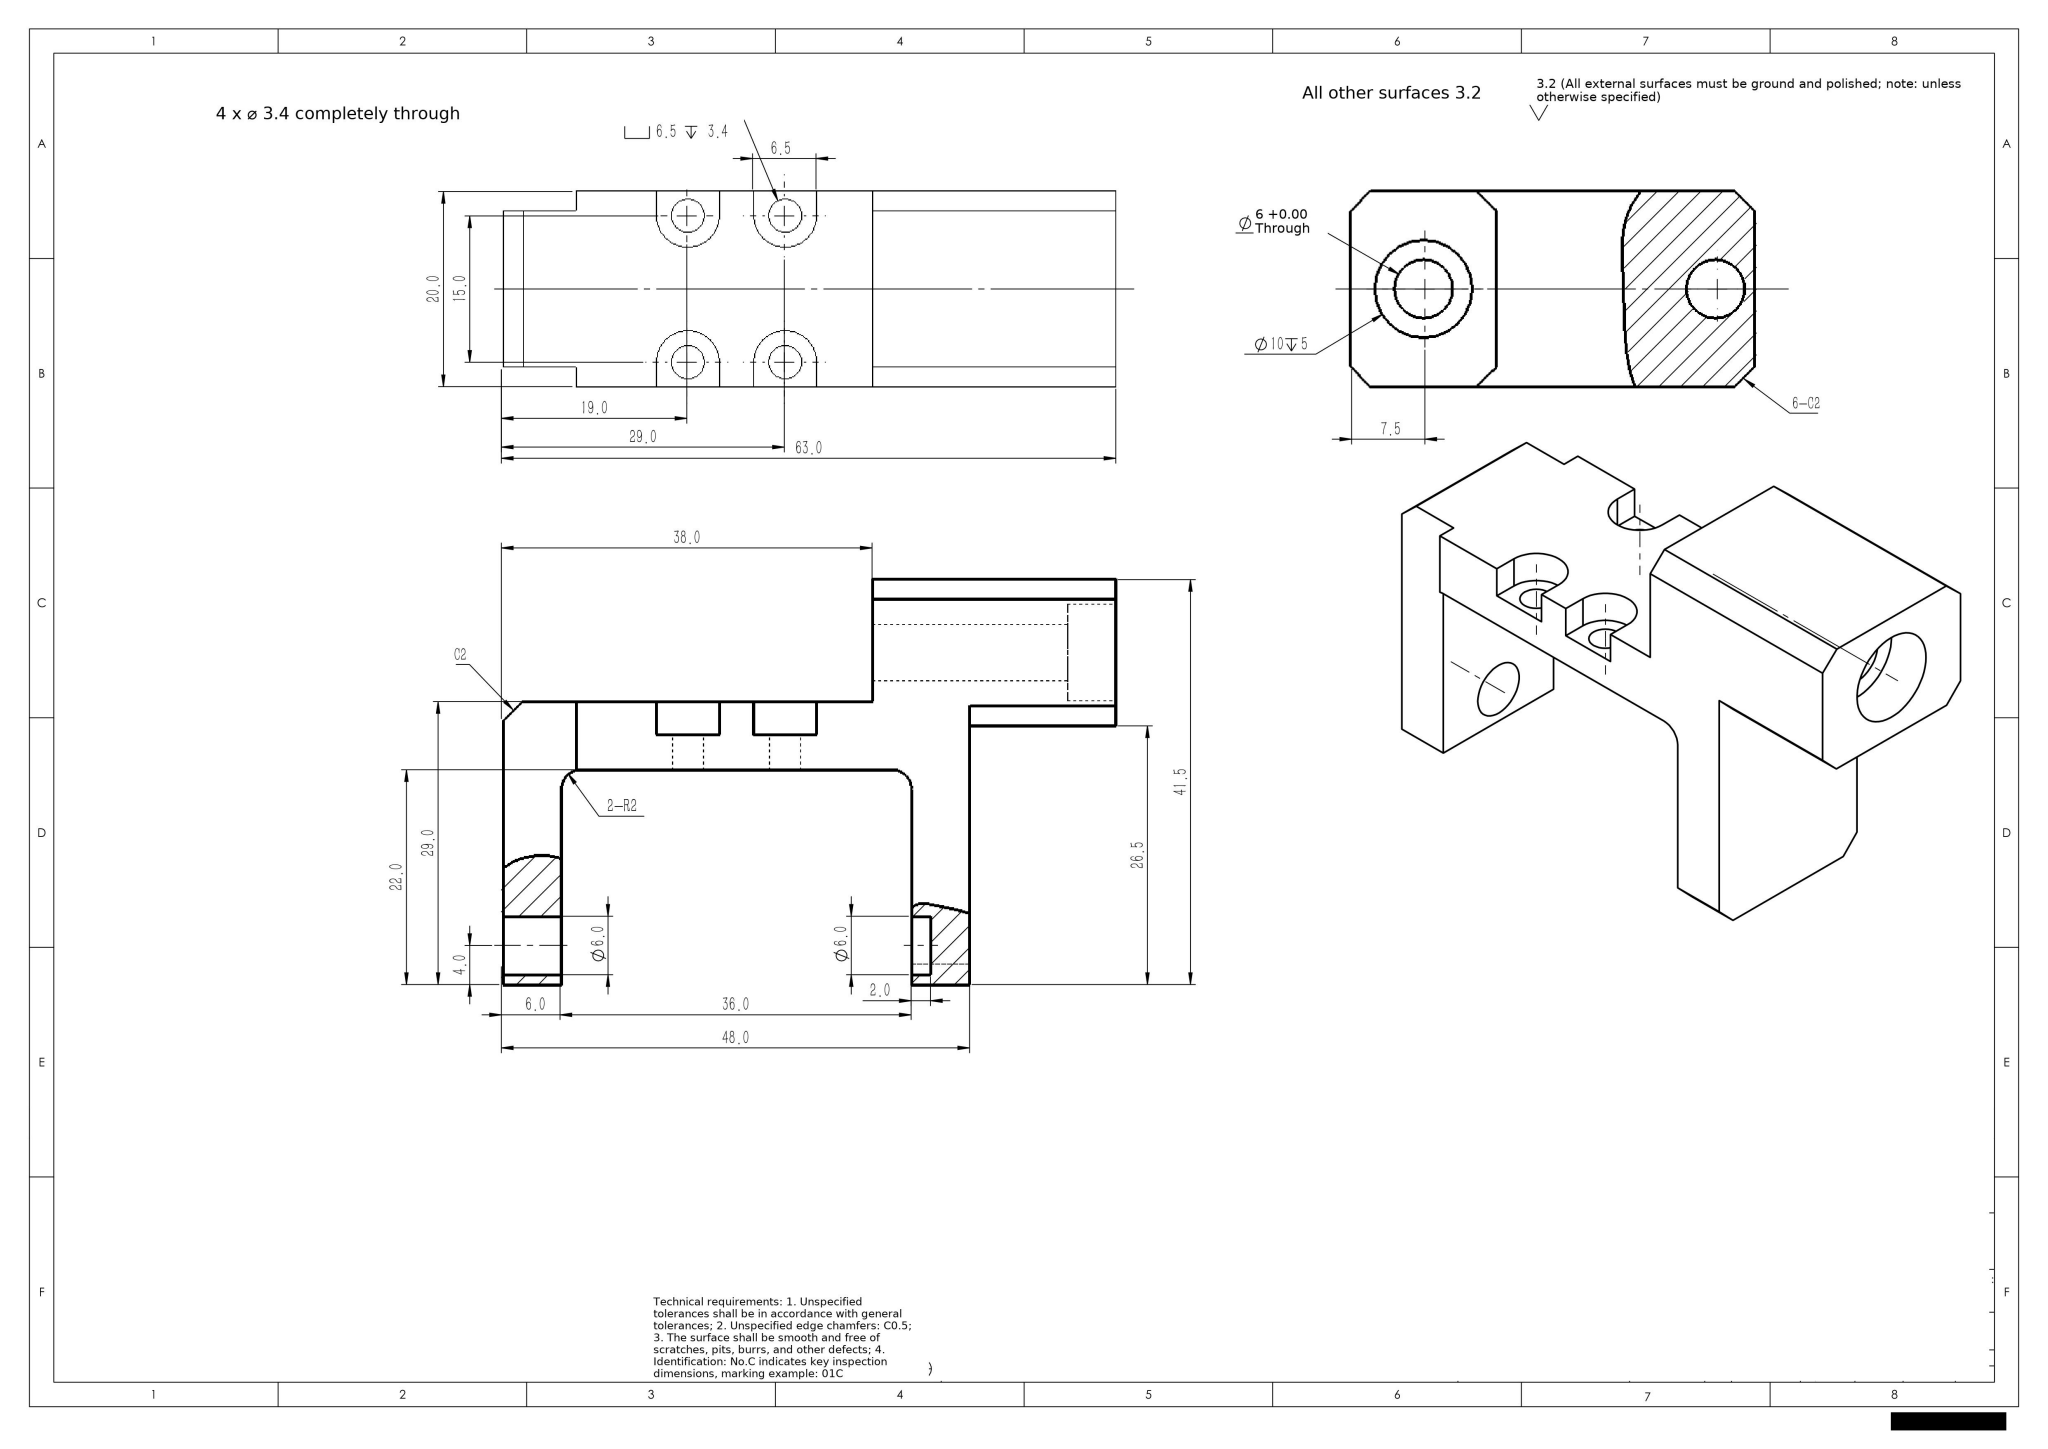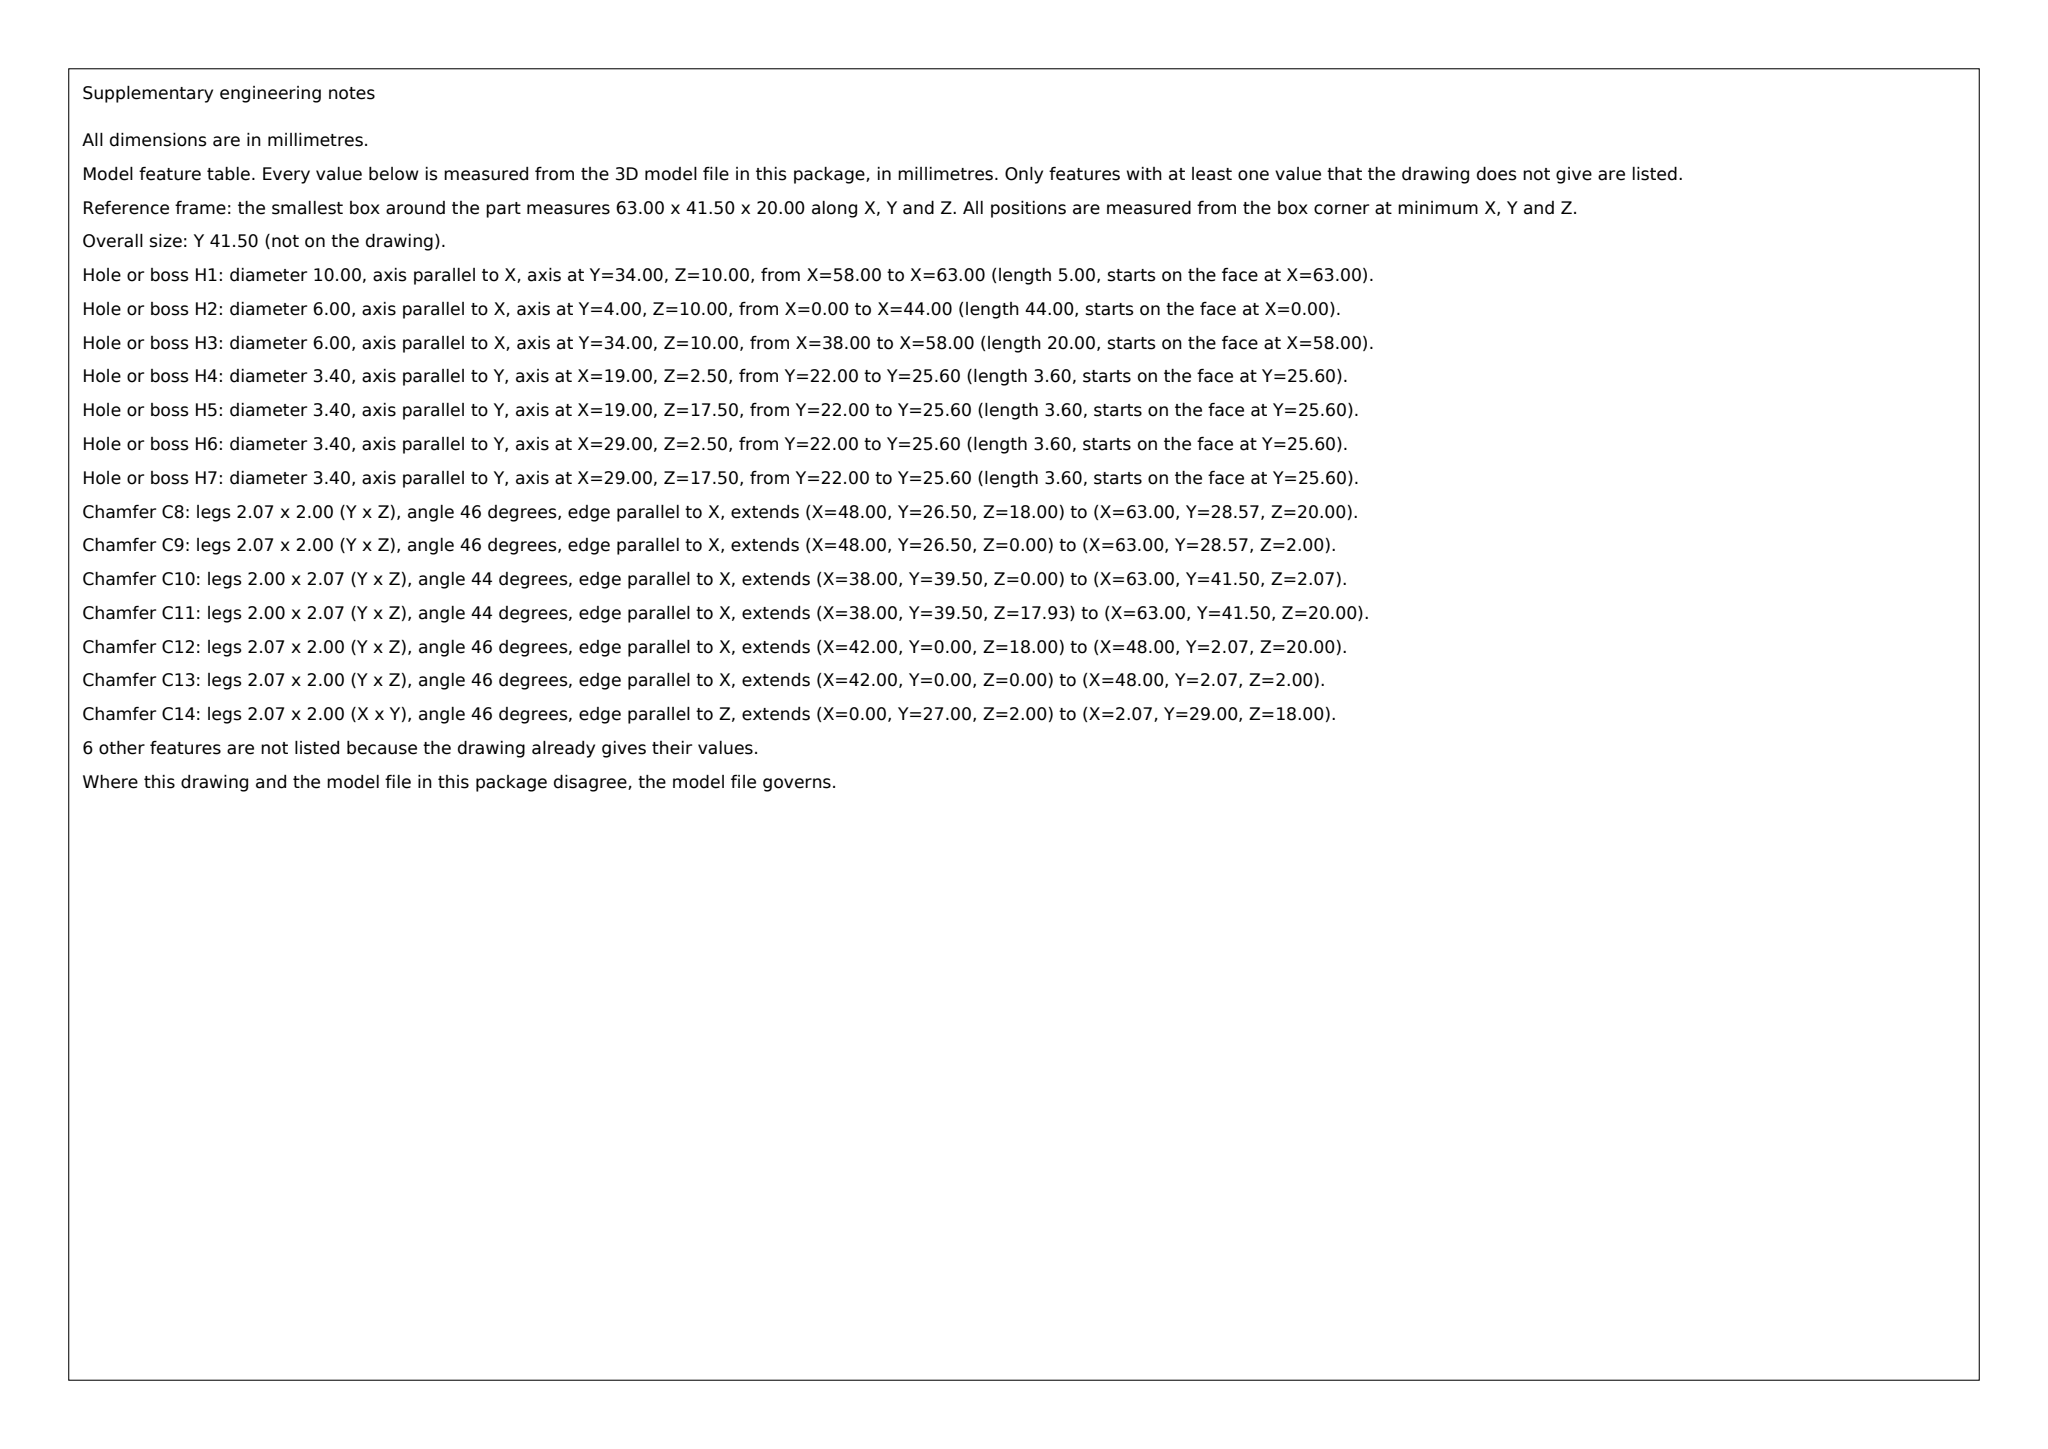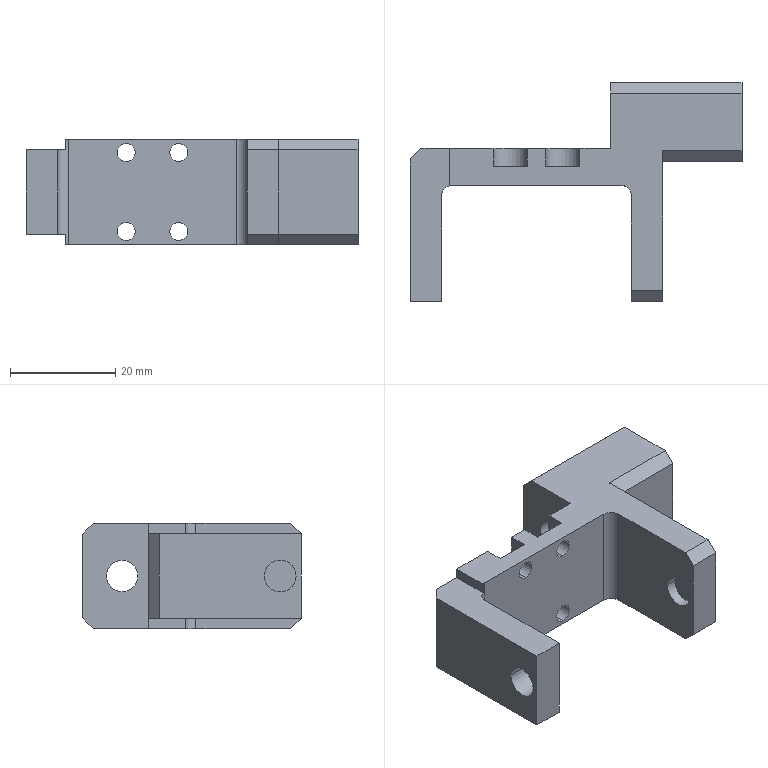Part | SolidWorks | mm | 1 solid | 63 faces | box 63 x 41.5 x 20 mm | volume 16308 mm3 | plane 39 | cylinder 24 | commonest cylinder face diameters 3.4 x8 6.5 x6 6 x6 10 x2 4 x2
build123d program:
from build123d import *
from OCP.BRepFilletAPI import BRepFilletAPI_MakeChamfer

# Parameters (mm, degrees)
SKETCH1_W                                       = 48
SKETCH1_H                                       = 20
BOSS_EXTRUDE1_DEPTH                             = 41.5
SKETCH4_W                                       = 36
SKETCH4_H                                       = 22
CUT_EXTRUDE3_DEPTH                              = 52.945
SKETCH5_W                                       = 38
SKETCH5_H                                       = 12.5
CUT_EXTRUDE4_DEPTH                              = 52.945
SKETCH10_W                                      = 15
SKETCH10_H                                      = 15
BOSS_EXTRUDE2_DEPTH                             = 20
SKETCH2_R                                       = 5
CUT_EXTRUDE1_DEPTH                              = 5
SKETCH3_R                                       = 3
CUT_EXTRUDE2_DEPTH                              = 73.016
SKETCH9_R                                       = 3
CUT_EXTRUDE6_DEPTH                              = 62.305
M3_HEX_SOCKET_HEAD_CAP_SCREW_CBORE1_D           = 3.4
M3_HEX_SOCKET_HEAD_CAP_SCREW_CBORE1_CBORE_D     = 6.5
M3_HEX_SOCKET_HEAD_CAP_SCREW_CBORE1_CBORE_DEPTH = 3.4
SKETCH11_W                                      = 6.5
SKETCH11_H                                      = 2.5
CUT_EXTRUDE7_DEPTH                              = 3.4
SKETCH12_W                                      = 9.952
SKETCH12_H                                      = 4.109
SKETCH12_H_2                                    = 3.368
CUT_EXTRUDE8_DEPTH                              = 50.619
FILLET2_R                                       = 2
CHAMFER2_SIZE                                   = 2
CHAMFER2_SIZE2                                  = 2.071


with BuildPart() as part:
    # Sketch1 → Boss-Extrude1 (new body)
    with BuildSketch(Plane(origin=(0, 0, 0), x_dir=(1, 0, 0), z_dir=(0, 1, 0))):
        Rectangle(SKETCH1_W, SKETCH1_H)
    extrude(amount=BOSS_EXTRUDE1_DEPTH)

    # Sketch4 → Cut-Extrude3 (cut, through all)
    with BuildSketch(Plane.XY.offset(10)):
        with Locations((0, 11)):
            Rectangle(SKETCH4_W, SKETCH4_H)
    extrude(amount=-CUT_EXTRUDE3_DEPTH, mode=Mode.SUBTRACT)

    # Sketch5 → Cut-Extrude4 (cut, through all)
    with BuildSketch(Plane.XY.offset(10)):
        with Locations((-5, 35.25)):
            Rectangle(SKETCH5_W, SKETCH5_H)
    extrude(amount=-CUT_EXTRUDE4_DEPTH, mode=Mode.SUBTRACT)

    # Sketch10 → Boss-Extrude2 (add)
    with BuildSketch(Plane(origin=(0, 0, -10), x_dir=(-1, 0, 0), z_dir=(0, 0, -1))):
        with Locations((-31.5, 34)):
            Rectangle(SKETCH10_W, SKETCH10_H)
    extrude(amount=-BOSS_EXTRUDE2_DEPTH)

    # Sketch2 → Cut-Extrude1 (cut)
    with BuildSketch(Plane(origin=(39, 0, 0), x_dir=(0, 0, -1), z_dir=(1, 0, 0))):
        with Locations((0, 34)):
            Circle(SKETCH2_R)
    extrude(amount=-CUT_EXTRUDE1_DEPTH, mode=Mode.SUBTRACT)

    # Sketch3 → Cut-Extrude2 (cut, through all)
    with BuildSketch(Plane(origin=(34, 0, 0), x_dir=(0, 0, -1), z_dir=(1, 0, 0))):
        with Locations((0, 34)):
            Circle(SKETCH3_R)
    extrude(amount=-CUT_EXTRUDE2_DEPTH, mode=Mode.SUBTRACT)

    # Sketch9 → Cut-Extrude6 (cut, through all)
    with BuildSketch(Plane.ZY.offset(-20)):
        with Locations(Location((0, 4, 0), (0, 0, 90))):
            Circle(SKETCH9_R)
    extrude(amount=CUT_EXTRUDE6_DEPTH, mode=Mode.SUBTRACT)

    # M3 Hex Socket Head Cap Screw CBORE1 (through all)
    with Locations(Plane(origin=(0, 29, 0), x_dir=(1, 0, 0), z_dir=(0, 1, 0))):
        with Locations((-5, -7.5), (-5, 7.5), (5, 7.5), (5, -7.5)):
            CounterBoreHole(M3_HEX_SOCKET_HEAD_CAP_SCREW_CBORE1_D / 2, M3_HEX_SOCKET_HEAD_CAP_SCREW_CBORE1_CBORE_D / 2, M3_HEX_SOCKET_HEAD_CAP_SCREW_CBORE1_CBORE_DEPTH)

    # Sketch11 → Cut-Extrude7 (cut)
    with BuildSketch(Plane(origin=(0, 29, 0), x_dir=(1, 0, 0), z_dir=(0, 1, 0))):
        with Locations((-5, 8.75)):
            Rectangle(SKETCH11_W, SKETCH11_H)
        with Locations((5, 8.75)):
            Rectangle(SKETCH11_W, SKETCH11_H)
        with Locations((5, -8.75)):
            Rectangle(SKETCH11_W, SKETCH11_H)
        with Locations((-5, -8.75)):
            Rectangle(SKETCH11_W, SKETCH11_H)
    extrude(amount=-CUT_EXTRUDE7_DEPTH, mode=Mode.SUBTRACT)

    # Sketch12 → Cut-Extrude8 (cut, through all)
    with BuildSketch(Plane(origin=(0, 29, 0), x_dir=(1, 0, 0), z_dir=(0, 1, 0))):
        with Locations((-21.476, 10.055)):
            Rectangle(SKETCH12_W, SKETCH12_H)
        with Locations((-21.476, -9.684)):
            Rectangle(SKETCH12_W, SKETCH12_H_2)
    extrude(amount=-CUT_EXTRUDE8_DEPTH, mode=Mode.SUBTRACT)

    # Fillet2
    fillet2_edges = [part.edges().sort_by_distance(p)[0] for p in [
        (-18, 22, 0),
        (18, 22, 0),
    ]]
    fillet(fillet2_edges, radius=FILLET2_R)

    # Chamfer2: one chamfer whose edges measure the first distance from different faces: ONE call of the kernel's chamfer builder (chamfer() names one face for all edges)
    chamfer2_edges_1 = [part.edges().sort_by_distance(p)[0] for p in [
        (21, 0, 10),
        (21, 0, -10),
    ]]
    chamfer2_side_1 = [part.faces().sort_by_distance(p)[0] for p in [
        (21, 0, 0),
    ]]
    chamfer2_edges_2 = [part.edges().sort_by_distance(p)[0] for p in [
        (-24, 29, 0),
    ]]
    chamfer2_side_2 = [part.faces().sort_by_distance(p)[0] for p in [
        (-24, 15.181, 0),
    ]]
    chamfer2_edges_3 = [part.edges().sort_by_distance(p)[0] for p in [
        (26.5, 41.5, 10),
    ]]
    chamfer2_side_3 = [part.faces().sort_by_distance(p)[0] for p in [
        (18.434, 27.071, 10),
    ]]
    chamfer2_edges_4 = [part.edges().sort_by_distance(p)[0] for p in [
        (31.5, 26.5, -10),
        (31.5, 26.5, 10),
    ]]
    chamfer2_side_4 = [part.faces().sort_by_distance(p)[0] for p in [
        (31.5, 26.5, 0),
    ]]
    chamfer2_edges_5 = [part.edges().sort_by_distance(p)[0] for p in [
        (26.5, 41.5, -10),
    ]]
    chamfer2_side_5 = [part.faces().sort_by_distance(p)[0] for p in [
        (18.434, 27.071, -10),
    ]]
    chamfer2 = BRepFilletAPI_MakeChamfer(part.part.solid().wrapped)
    for e in chamfer2_edges_1:
        chamfer2.Add(CHAMFER2_SIZE, CHAMFER2_SIZE2, e.wrapped, chamfer2_side_1[0].wrapped)  # the first distance lies on this face
    for e in chamfer2_edges_2:
        chamfer2.Add(CHAMFER2_SIZE, CHAMFER2_SIZE2, e.wrapped, chamfer2_side_2[0].wrapped)  # the first distance lies on this face
    for e in chamfer2_edges_3:
        chamfer2.Add(CHAMFER2_SIZE, CHAMFER2_SIZE2, e.wrapped, chamfer2_side_3[0].wrapped)  # the first distance lies on this face
    for e in chamfer2_edges_4:
        chamfer2.Add(CHAMFER2_SIZE, CHAMFER2_SIZE2, e.wrapped, chamfer2_side_4[0].wrapped)  # the first distance lies on this face
    for e in chamfer2_edges_5:
        chamfer2.Add(CHAMFER2_SIZE, CHAMFER2_SIZE2, e.wrapped, chamfer2_side_5[0].wrapped)  # the first distance lies on this face
    add(Compound.cast(chamfer2.Shape()), mode=Mode.REPLACE)


solid = part.part